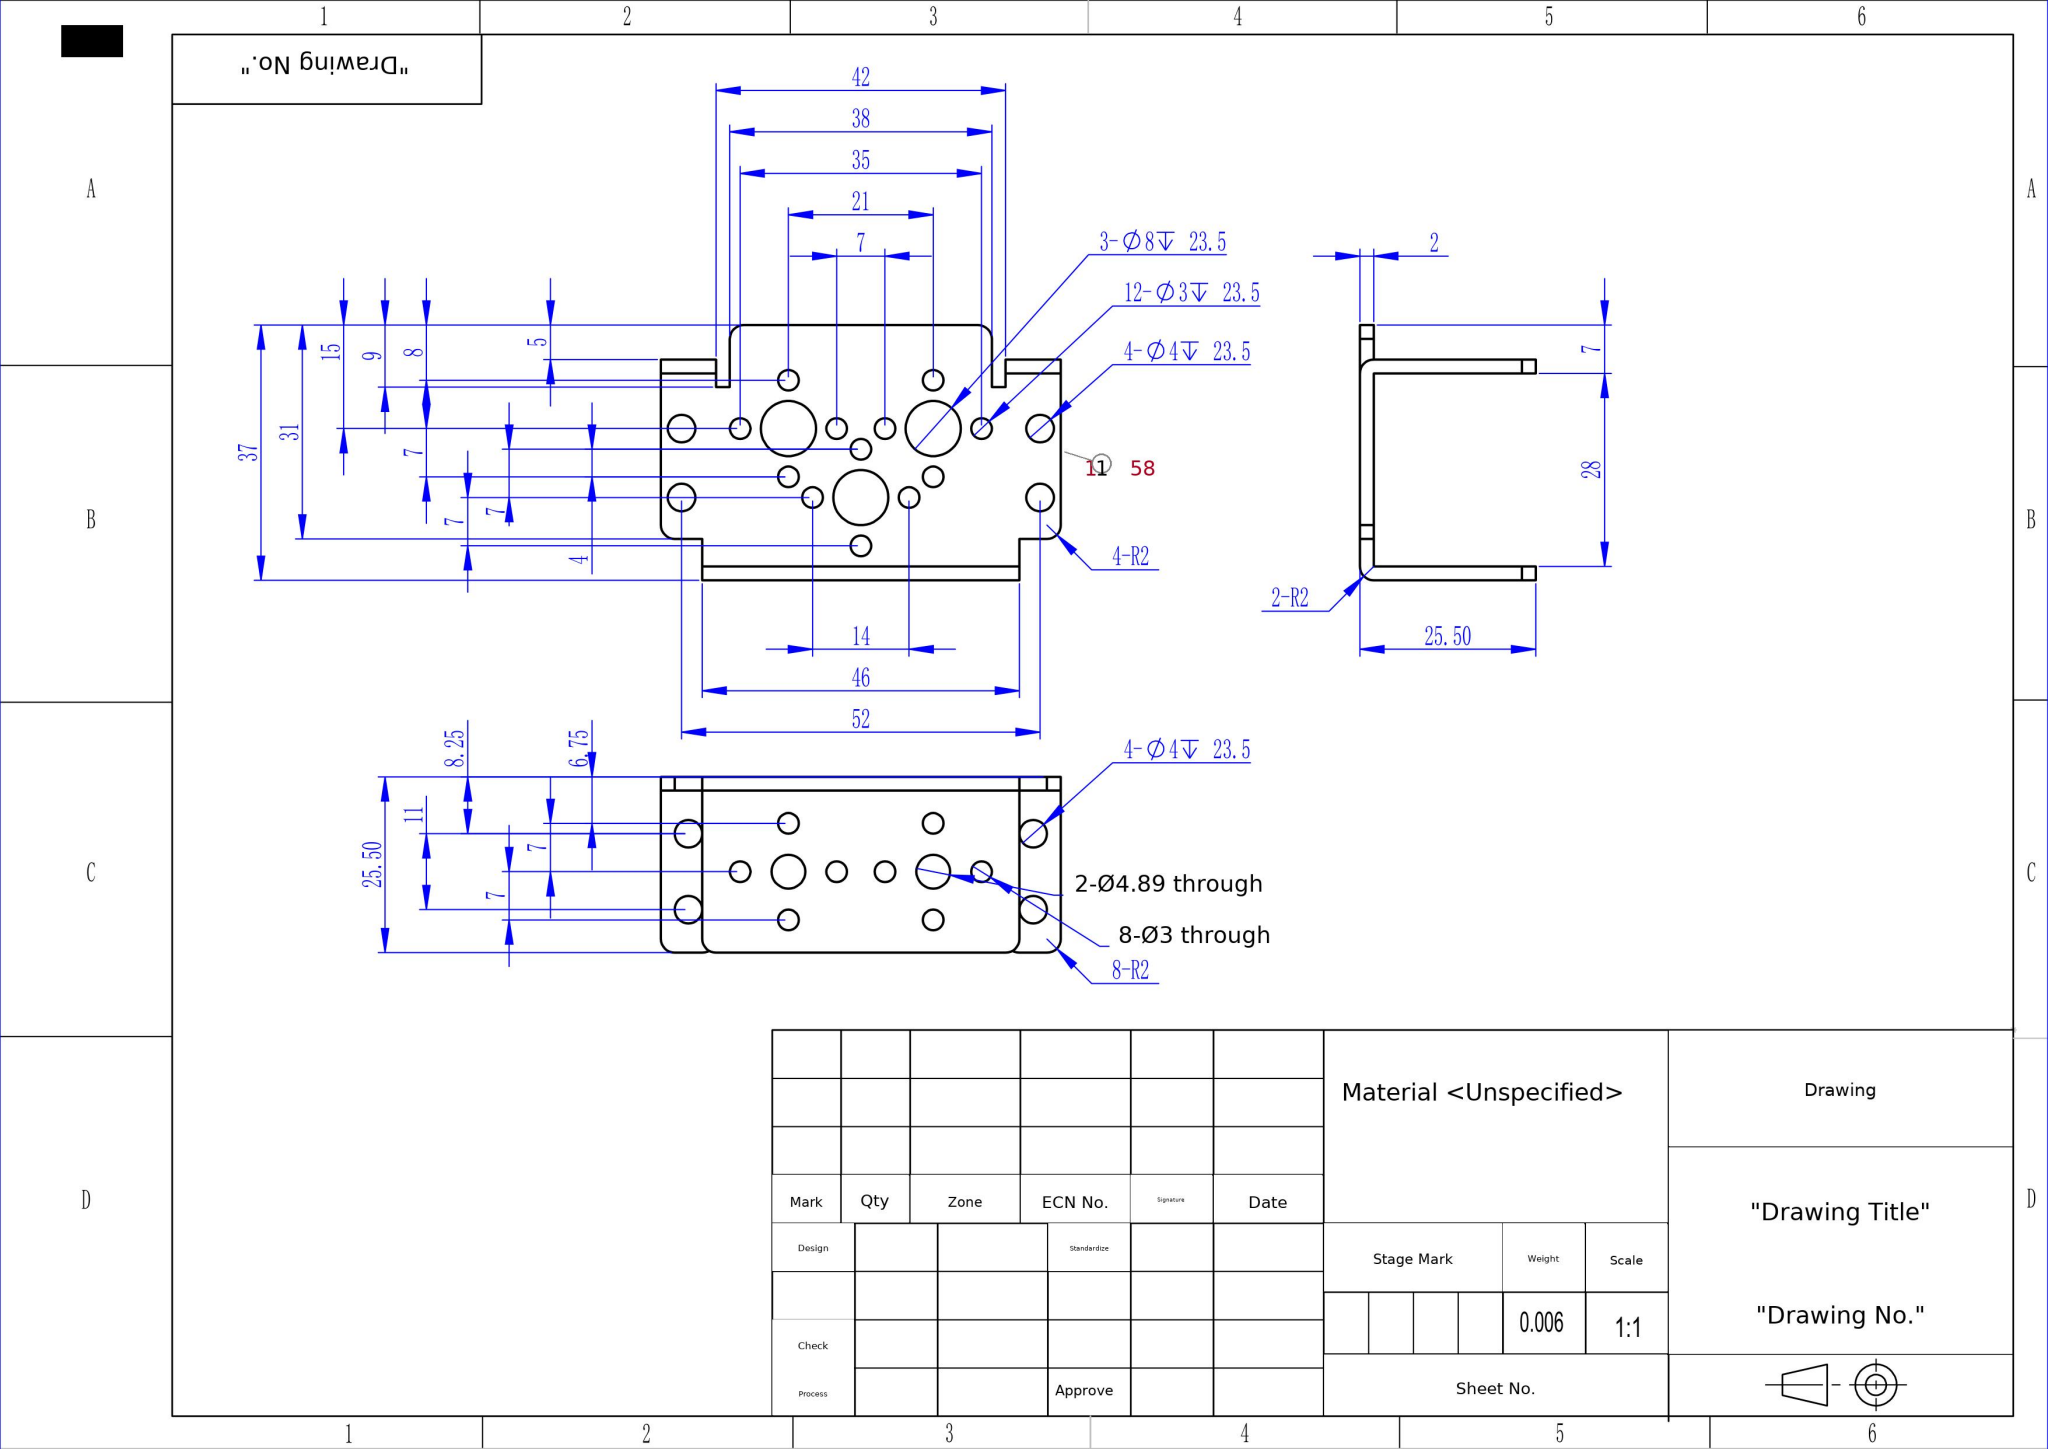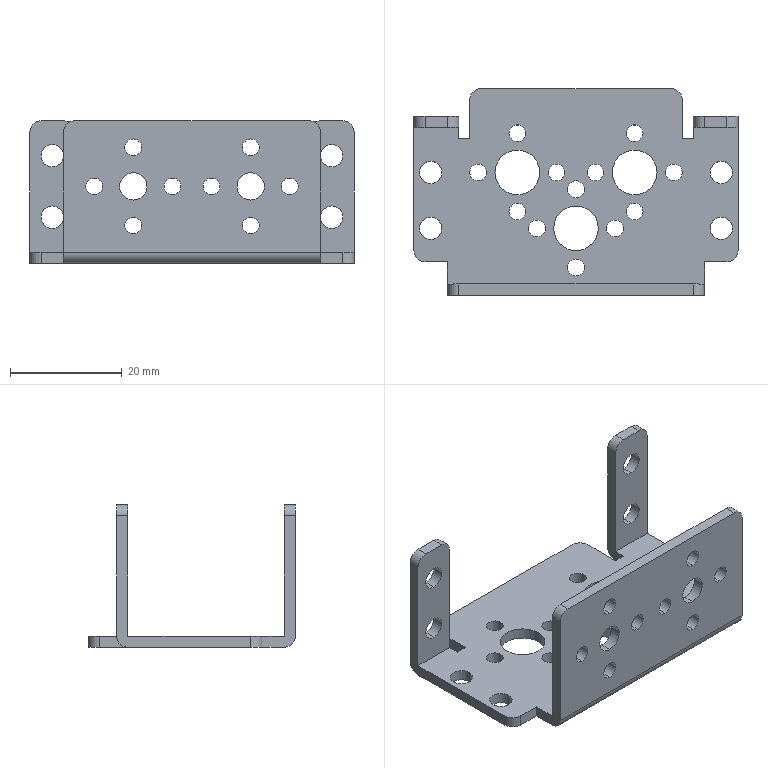Part | SolidWorks | mm | 1 solid | 103 faces | box 58 x 37 x 25.5 mm | volume 5899 mm3 | cylinder 79 | plane 24 | commonest cylinder face diameters 3 x40 4 x29 8 x6 4.894 x4
build123d program:
from build123d import *

# Parameters (mm, degrees)
SKETCH3_W           = 58
SKETCH3_H           = 37
BOSS_EXTRUDE1_DEPTH = 2
SKETCH4_W           = 58
SKETCH4_H           = 2
BOSS_EXTRUDE2_DEPTH = 23.5
SKETCH5_W           = 8
SKETCH5_H           = 2
BOSS_EXTRUDE3_DEPTH = 23.5
LPATTERN1_COUNT     = 2
LPATTERN1_PITCH     = 50
SKETCH6_W           = 6
SKETCH6_H           = 6
CUT_EXTRUDE1_DEPTH  = 44.951
LPATTERN2_COUNT     = 2
LPATTERN2_PITCH     = 52
CUT_EXTRUDE2_DEPTH  = 23.5
CUT_EXTRUDE3_DEPTH  = 23.5
SKETCH9_R           = 2
SKETCH9_R_2         = 4
SKETCH9_R_3         = 1.5
CUT_EXTRUDE4_DEPTH  = 23.5
SKETCH11_R          = 2.447
SKETCH11_R_2        = 1.5
CUT_EXTRUDE5_DEPTH  = 53.925
FILLET1_R           = 2
SKETCH12_R          = 2
CUT_EXTRUDE6_DEPTH  = 23.5


with BuildPart() as part:
    # Sketch3 → Boss-Extrude1 (new body)
    with BuildSketch(Plane.XY):
        with Locations((-1.427, 2.798)):
            Rectangle(SKETCH3_W, SKETCH3_H)
    extrude(amount=BOSS_EXTRUDE1_DEPTH)

    # Sketch4 → Boss-Extrude2 (add)
    with BuildSketch(Plane.XY.offset(2)):
        with Locations((-1.427, -14.702)):
            Rectangle(SKETCH4_W, SKETCH4_H)
    extrude(amount=BOSS_EXTRUDE2_DEPTH)

    # Sketch5 → Boss-Extrude3 (add)
    with BuildSketch(Plane.XY.offset(2)):
        with Locations((-26.427, 15.298)):
            Rectangle(SKETCH5_W, SKETCH5_H)
    boss_extrude3 = extrude(amount=BOSS_EXTRUDE3_DEPTH)

    # LPattern1: Boss-Extrude3 ×2
    with Locations(*[(i * LPATTERN1_PITCH, 0, 0) for i in range(1, LPATTERN1_COUNT)]):
        add(boss_extrude3)

    # Sketch6 → Cut-Extrude1 (cut, symmetric)
    with BuildSketch(Plane.XY.offset(2)):
        with Locations((-27.427, -12.702)):
            Rectangle(SKETCH6_W, SKETCH6_H)
    cut_extrude1 = extrude(amount=CUT_EXTRUDE1_DEPTH, both=True, mode=Mode.SUBTRACT)

    # LPattern2: Cut-Extrude1 ×2
    with Locations(*[(i * LPATTERN2_PITCH, 0, 0) for i in range(1, LPATTERN2_COUNT)]):
        add(cut_extrude1, mode=Mode.SUBTRACT)

    # Sketch7 → Cut-Extrude2 (cut)
    with BuildSketch(Plane.XY.offset(2)):
        Polygon((-30.427, 21.298), (-30.427, 16.298), (-22.427, 16.298), (-22.427, 14.298), (-22.427, 12.298), (-20.427, 12.298), (-20.427, 21.298), align=None)
    extrude(amount=-CUT_EXTRUDE2_DEPTH, mode=Mode.SUBTRACT)

    # Sketch8 → Cut-Extrude3 (cut)
    with BuildSketch(Plane.XY.offset(2)):
        Polygon((27.573, 16.298), (27.573, 21.298), (17.573, 21.298), (17.573, 12.298), (19.573, 12.298), (19.573, 16.298), align=None)
    extrude(amount=-CUT_EXTRUDE3_DEPTH, mode=Mode.SUBTRACT)

    # Sketch9 → Cut-Extrude4 (cut)
    with BuildSketch(Plane.XY.offset(2)):
        with Locations((-27.427, 6.298)):
            Circle(SKETCH9_R)
        with Locations((-27.427, -3.702)):
            Circle(SKETCH9_R)
        with Locations((-11.927, 6.298)):
            Circle(SKETCH9_R_2)
        with Locations((-1.427, -3.702)):
            Circle(SKETCH9_R_2)
        with Locations((-1.427, 3.298)):
            Circle(SKETCH9_R_3)
        with Locations((-1.427, -10.702)):
            Circle(SKETCH9_R_3)
        with Locations((-11.927, -0.7021)):
            Circle(SKETCH9_R_3)
        with Locations((-11.927, 13.298)):
            Circle(SKETCH9_R_3)
        with Locations((-18.927, 6.298)):
            Circle(SKETCH9_R_3)
        with Locations((-4.927, 6.298)):
            Circle(SKETCH9_R_3)
        with Locations((-8.427, -3.702)):
            Circle(SKETCH9_R_3)
        with Locations((5.573, -3.702)):
            Circle(SKETCH9_R_3)
        with Locations((9.073, 13.298)):
            Circle(SKETCH9_R_3)
        with Locations((2.073, 6.298)):
            Circle(SKETCH9_R_3)
        with Locations((9.073, -0.7021)):
            Circle(SKETCH9_R_3)
        with Locations((9.073, 6.298)):
            Circle(SKETCH9_R_2)
        with Locations((16.073, 6.298)):
            Circle(SKETCH9_R_3)
        with Locations((24.573, -3.702)):
            Circle(SKETCH9_R)
        with Locations((24.573, 6.298)):
            Circle(SKETCH9_R)
    extrude(amount=-CUT_EXTRUDE4_DEPTH, mode=Mode.SUBTRACT)

    # Sketch11 → Cut-Extrude5 (cut, through all)
    with BuildSketch(Plane(origin=(0, -13.702, 0), x_dir=(1, 0, 0), z_dir=(0, 1, 0))):
        with Locations(Location((-11.927, -13.75, 0), (0, 0, 270))):
            Circle(SKETCH11_R)
        with Locations(Location((-18.927, -13.75, 0), (0, 0, 270))):
            Circle(SKETCH11_R_2)
        with Locations(Location((-11.927, -20.75, 0), (0, 0, 270))):
            Circle(SKETCH11_R_2)
        with Locations(Location((-4.927, -13.75, 0), (0, 0, 270))):
            Circle(SKETCH11_R_2)
        with Locations(Location((-11.927, -6.75, 0), (0, 0, 270))):
            Circle(SKETCH11_R_2)
        with Locations(Location((9.073, -20.75, 0), (0, 0, 90))):
            Circle(SKETCH11_R_2)
        with Locations(Location((2.073, -13.75, 0), (0, 0, 90))):
            Circle(SKETCH11_R_2)
        with Locations(Location((9.073, -6.75, 0), (0, 0, 90))):
            Circle(SKETCH11_R_2)
        with Locations(Location((9.073, -13.75, 0), (0, 0, 90))):
            Circle(SKETCH11_R)
        with Locations(Location((16.073, -13.75, 0), (0, 0, 90))):
            Circle(SKETCH11_R_2)
    extrude(amount=-CUT_EXTRUDE5_DEPTH, mode=Mode.SUBTRACT)

    # Fillet1
    fillet1_edges = [part.edges().sort_by_distance(p)[0] for p in [
        (-1.427, -15.702, 0),
        (-30.427, -9.702, 1),
        (27.573, -9.702, 1),
        (-20.427, 21.298, 1),
        (17.573, 21.298, 1),
        (23.573, 16.298, 0),
        (-26.427, 16.298, 0),
        (27.573, 15.298, 25.5),
        (19.573, 15.298, 25.5),
        (21.573, -14.702, 25.5),
        (-24.427, -14.702, 25.5),
        (-22.427, 15.298, 25.5),
        (-30.427, 15.298, 25.5),
    ]]
    fillet(fillet1_edges, radius=FILLET1_R)

    # Sketch12 → Cut-Extrude6 (cut)
    with BuildSketch(Plane(origin=(0, 16.298, 0), x_dir=(1, 0, 0), z_dir=(0, 1, 0))):
        with Locations(Location((-26.427, -19.25, 0), (0, 0, 270))):
            Circle(SKETCH12_R)
        with Locations(Location((-26.427, -8.25, 0), (0, 0, 270))):
            Circle(SKETCH12_R)
        with Locations(Location((23.573, -19.25, 0), (0, 0, 270))):
            Circle(SKETCH12_R)
        with Locations(Location((23.573, -8.25, 0), (0, 0, 270))):
            Circle(SKETCH12_R)
    extrude(amount=-CUT_EXTRUDE6_DEPTH, mode=Mode.SUBTRACT)


solid = part.part